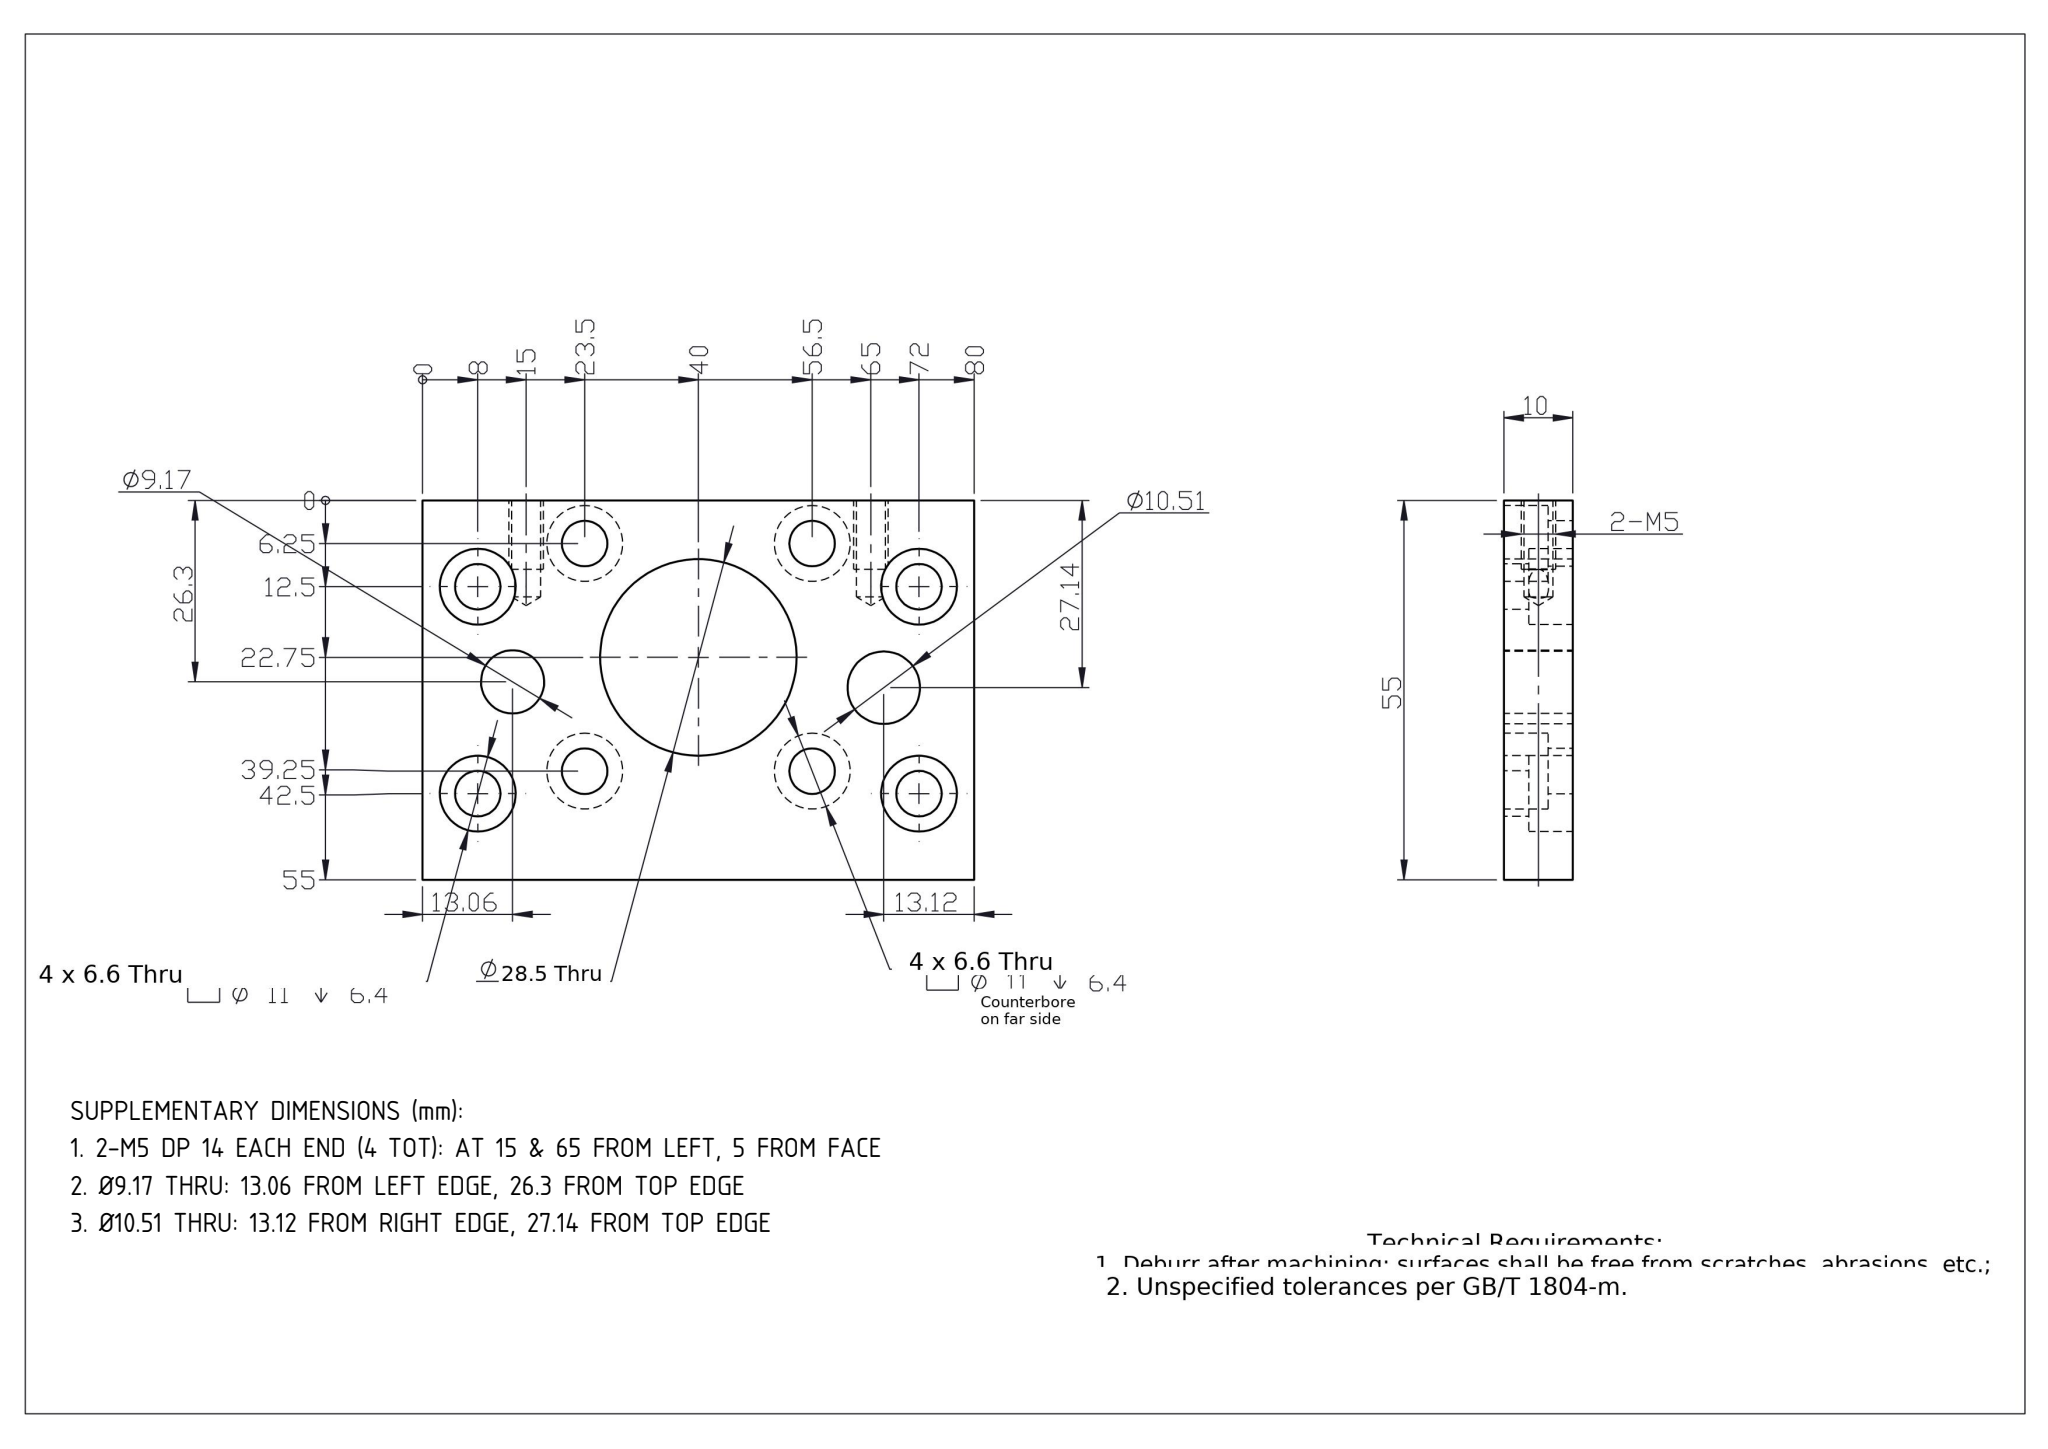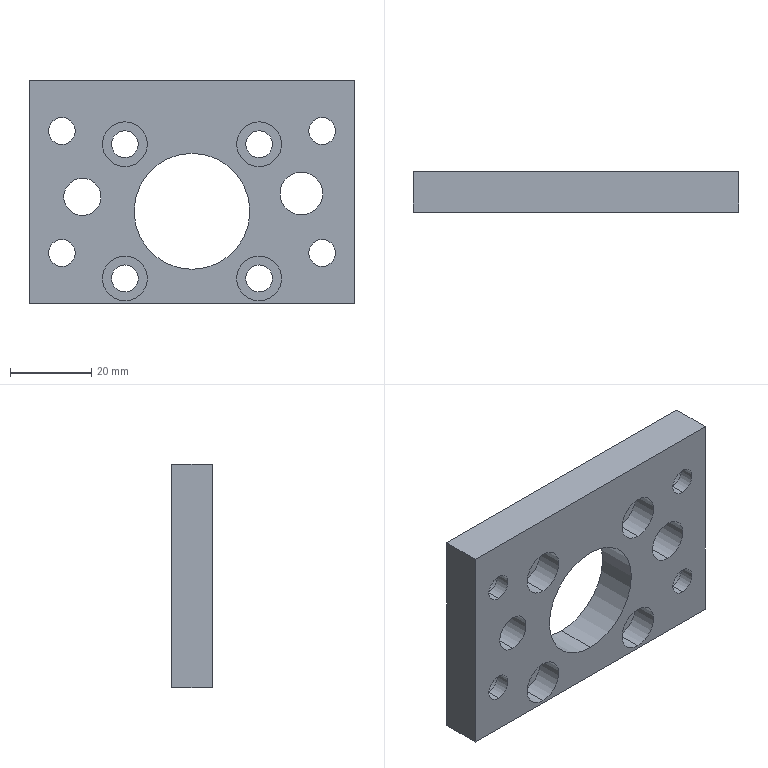Part | SolidWorks | mm | 1 solid | 60 faces | box 80 x 10 x 55 mm | volume 29848 mm3 | cylinder 42 | plane 14 | cone 4 | commonest cylinder face diameters 11 x16 6.6 x16 4.2 x4 9.17 x2 10.512 x2 28.5 x2
build123d program:
from build123d import *

# Parameters (mm, degrees)
SKETCH1_W                                       = 80
SKETCH1_H                                       = 10
BOSS_EXTRUDE1_DEPTH                             = 55
M6_HEX_SOCKET_HEAD_CAP_SCREW_CBORE1_D           = 6.6
M6_HEX_SOCKET_HEAD_CAP_SCREW_CBORE1_CBORE_D     = 11
M6_HEX_SOCKET_HEAD_CAP_SCREW_CBORE1_CBORE_DEPTH = 6.4
M5_TAPPED_HOLE1_D                               = 4.2
M5_TAPPED_HOLE1_DEPTH                           = 14
M5_TAPPED_HOLE1_TIP                             = 1.262
SKETCH6_R                                       = 14.25
CUT_EXTRUDE1_DEPTH                              = 98.596
M6_HEX_SOCKET_HEAD_CAP_SCREW_CBORE2_D           = 6.6
M6_HEX_SOCKET_HEAD_CAP_SCREW_CBORE2_CBORE_D     = 11
M6_HEX_SOCKET_HEAD_CAP_SCREW_CBORE2_CBORE_DEPTH = 6.4
SKETCH9_R                                       = 4.585
SKETCH9_R_2                                     = 5.256
CUT_EXTRUDE2_DEPTH                              = 10


with BuildPart() as part:
    # Sketch1 → Boss-Extrude1 (new body)
    with BuildSketch(Plane.XY):
        with Locations((40, -5)):
            Rectangle(SKETCH1_W, SKETCH1_H)
    extrude(amount=BOSS_EXTRUDE1_DEPTH)

    # M6 Hex Socket Head Cap Screw CBORE1 (through all)
    with Locations(Plane(origin=(0, 0, 0), x_dir=(1, 0, 0), z_dir=(0, 1, 0))):
        with Locations((8, -12.5), (8, -42.5), (72, -42.5), (72, -12.5)):
            CounterBoreHole(M6_HEX_SOCKET_HEAD_CAP_SCREW_CBORE1_D / 2, M6_HEX_SOCKET_HEAD_CAP_SCREW_CBORE1_CBORE_D / 2, M6_HEX_SOCKET_HEAD_CAP_SCREW_CBORE1_CBORE_DEPTH)

    # M5 Tapped Hole1
    with Locations(Plane(origin=(0, 0, 0), x_dir=(-1, 0, 0), z_dir=(0, 0, -1))):
        with Locations((-65, -5), (-15, -5)):
            Hole(M5_TAPPED_HOLE1_D / 2, depth=M5_TAPPED_HOLE1_DEPTH)
            with Locations((0, 0, -(M5_TAPPED_HOLE1_DEPTH + M5_TAPPED_HOLE1_TIP / 2))):  # 118° drill point
                Cone(0, M5_TAPPED_HOLE1_D / 2, M5_TAPPED_HOLE1_TIP, mode=Mode.SUBTRACT)

    # Sketch6 → Cut-Extrude1 (cut, through all)
    with BuildSketch(Plane(origin=(0, 0, 0), x_dir=(1, 0, 0), z_dir=(0, 1, 0))):
        with Locations(Location((40, -22.75, 0), (0, 0, 270))):
            Circle(SKETCH6_R)
    extrude(amount=-CUT_EXTRUDE1_DEPTH, mode=Mode.SUBTRACT)

    # M6 Hex Socket Head Cap Screw CBORE2 (through all)
    with Locations(Plane(origin=(0, -10, 0), x_dir=(-1, 0, 0), z_dir=(0, -1, 0))):
        with Locations((-56.5, -6.25), (-23.5, -6.25), (-23.5, -39.25), (-56.5, -39.25)):
            CounterBoreHole(M6_HEX_SOCKET_HEAD_CAP_SCREW_CBORE2_D / 2, M6_HEX_SOCKET_HEAD_CAP_SCREW_CBORE2_CBORE_D / 2, M6_HEX_SOCKET_HEAD_CAP_SCREW_CBORE2_CBORE_DEPTH)

    # Sketch9 → Cut-Extrude2 (cut)
    with BuildSketch(Plane(origin=(0, 0, 0), x_dir=(1, 0, 0), z_dir=(0, 1, 0))):
        with Locations(Location((13.055, -26.302, 0), (0, 0, 270))):
            Circle(SKETCH9_R)
        with Locations(Location((66.885, -27.141, 0), (0, 0, 270))):
            Circle(SKETCH9_R_2)
    extrude(amount=-CUT_EXTRUDE2_DEPTH, mode=Mode.SUBTRACT)


solid = part.part